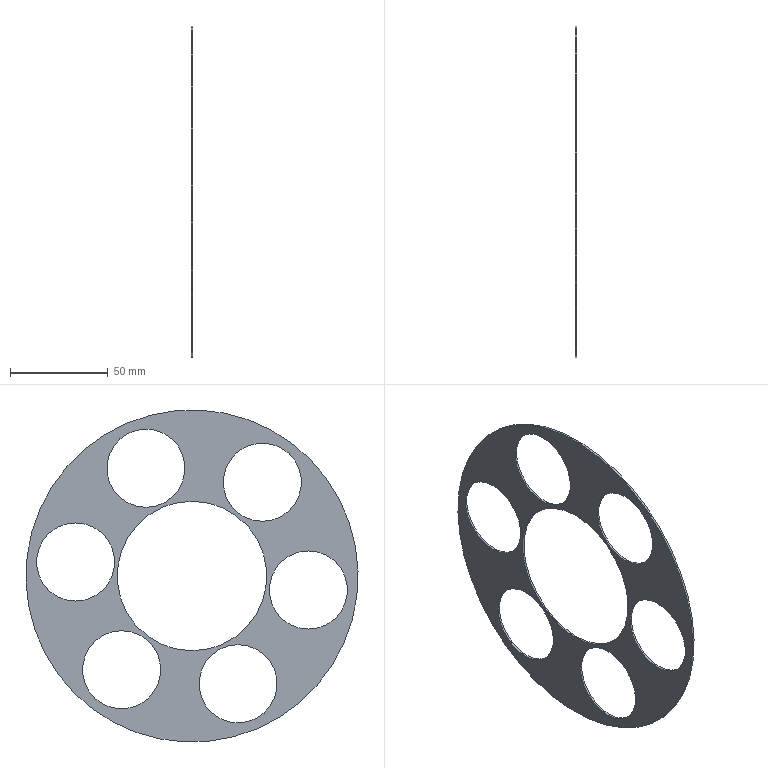Component | SolidWorks | 2018SOLIDWORKS1000000502-1 | 1 solid | 18 faces | box 1 x 170 x 170 mm | volume 10562 mm3 | cylinder 16 | plane 2 | commonest cylinder face diameters 40 x12 76.5 x2 170 x2 | material 201
STEP:
#1=COLOUR_RGB('',0.7922,0.8196,0.9333);
#2=FILL_AREA_STYLE_COLOUR('',#1);
#3=FILL_AREA_STYLE('',(#2));
#4=SURFACE_STYLE_FILL_AREA(#3);
#5=SURFACE_SIDE_STYLE('',(#4));
#6=SURFACE_STYLE_USAGE(.BOTH.,#5);
#7=PRESENTATION_STYLE_ASSIGNMENT((#6));
#8=CARTESIAN_POINT('',(0.3825,-4.408,10.134));
#9=VERTEX_POINT('',#8);
#10=CARTESIAN_POINT('',(0.3825,-5.972,9.946));
#11=VERTEX_POINT('',#10);
#12=CARTESIAN_POINT('',(0.3825,-5.19,10.04));
#13=DIRECTION('',(-1.,-0.,0.));
#14=DIRECTION('',(0.,-0.5999,0.8001));
#15=AXIS2_PLACEMENT_3D('',#12,#13,#14);
#16=CIRCLE('',#15,0.7874);
#17=EDGE_CURVE('',#9,#11,#16,.T.);
#18=ORIENTED_EDGE('',*,*,#17,.F.);
#19=CARTESIAN_POINT('',(0.3432,-4.408,10.134));
#20=VERTEX_POINT('',#19);
#21=CARTESIAN_POINT('',(0.3825,-4.408,10.134));
#22=DIRECTION('',(-1.,-0.,0.));
#23=VECTOR('',#22,39.37);
#24=LINE('',#21,#23);
#25=EDGE_CURVE('',#9,#20,#24,.T.);
#26=ORIENTED_EDGE('',*,*,#25,.T.);
#27=CARTESIAN_POINT('',(0.3432,-5.972,9.946));
#28=VERTEX_POINT('',#27);
#29=CARTESIAN_POINT('',(0.3432,-5.19,10.04));
#30=DIRECTION('',(-1.,-0.,0.));
#31=DIRECTION('',(0.,-0.5999,0.8001));
#32=AXIS2_PLACEMENT_3D('',#29,#30,#31);
#33=CIRCLE('',#32,0.7874);
#34=EDGE_CURVE('',#20,#28,#33,.T.);
#35=ORIENTED_EDGE('',*,*,#34,.T.);
#36=CARTESIAN_POINT('',(0.3825,-5.972,9.946));
#37=DIRECTION('',(-1.,-0.,0.));
#38=VECTOR('',#37,39.37);
#39=LINE('',#36,#38);
#40=EDGE_CURVE('',#11,#28,#39,.T.);
#41=ORIENTED_EDGE('',*,*,#40,.F.);
#42=EDGE_LOOP('',(#18,#26,#35,#41));
#43=FACE_OUTER_BOUND('',#42,.T.);
#44=CARTESIAN_POINT('',(0.3825,-5.19,10.04));
#45=DIRECTION('',(-1.,-0.,0.));
#46=DIRECTION('',(0.,-0.9928,-0.1195));
#47=AXIS2_PLACEMENT_3D('',#44,#45,#46);
#48=CYLINDRICAL_SURFACE('',#47,0.7874);
#49=ADVANCED_FACE('',(#43),#48,.F.);
#50=CARTESIAN_POINT('',(0.3825,-2.063,10.417));
#51=VERTEX_POINT('',#50);
#52=CARTESIAN_POINT('',(0.3825,-3.626,10.228));
#53=VERTEX_POINT('',#52);
#54=CARTESIAN_POINT('',(0.3825,-2.845,10.323));
#55=DIRECTION('',(-1.,-0.,0.));
#56=DIRECTION('',(0.,0.3929,0.9196));
#57=AXIS2_PLACEMENT_3D('',#54,#55,#56);
#58=CIRCLE('',#57,0.7874);
#59=EDGE_CURVE('',#51,#53,#58,.T.);
#60=ORIENTED_EDGE('',*,*,#59,.F.);
#61=CARTESIAN_POINT('',(0.3432,-2.063,10.417));
#62=VERTEX_POINT('',#61);
#63=CARTESIAN_POINT('',(0.3825,-2.063,10.417));
#64=DIRECTION('',(-1.,-0.,0.));
#65=VECTOR('',#64,39.37);
#66=LINE('',#63,#65);
#67=EDGE_CURVE('',#51,#62,#66,.T.);
#68=ORIENTED_EDGE('',*,*,#67,.T.);
#69=CARTESIAN_POINT('',(0.3432,-3.626,10.228));
#70=VERTEX_POINT('',#69);
#71=CARTESIAN_POINT('',(0.3432,-2.845,10.323));
#72=DIRECTION('',(-1.,-0.,0.));
#73=DIRECTION('',(0.,0.3929,0.9196));
#74=AXIS2_PLACEMENT_3D('',#71,#72,#73);
#75=CIRCLE('',#74,0.7874);
#76=EDGE_CURVE('',#62,#70,#75,.T.);
#77=ORIENTED_EDGE('',*,*,#76,.T.);
#78=CARTESIAN_POINT('',(0.3825,-3.626,10.228));
#79=DIRECTION('',(-1.,-0.,0.));
#80=VECTOR('',#79,39.37);
#81=LINE('',#78,#80);
#82=EDGE_CURVE('',#53,#70,#81,.T.);
#83=ORIENTED_EDGE('',*,*,#82,.F.);
#84=EDGE_LOOP('',(#60,#68,#77,#83));
#85=FACE_OUTER_BOUND('',#84,.T.);
#86=CARTESIAN_POINT('',(0.3825,-2.845,10.323));
#87=DIRECTION('',(-1.,-0.,0.));
#88=DIRECTION('',(0.,-0.9928,-0.1195));
#89=AXIS2_PLACEMENT_3D('',#86,#87,#88);
#90=CYLINDRICAL_SURFACE('',#89,0.7874);
#91=ADVANCED_FACE('',(#85),#90,.F.);
#92=CARTESIAN_POINT('',(0.3825,-0.6456,8.527));
#93=VERTEX_POINT('',#92);
#94=CARTESIAN_POINT('',(0.3825,-2.209,8.339));
#95=VERTEX_POINT('',#94);
#96=CARTESIAN_POINT('',(0.3825,-1.427,8.433));
#97=DIRECTION('',(-1.,-0.,0.));
#98=DIRECTION('',(-0.,0.9928,0.1195));
#99=AXIS2_PLACEMENT_3D('',#96,#97,#98);
#100=CIRCLE('',#99,0.7874);
#101=EDGE_CURVE('',#93,#95,#100,.T.);
#102=ORIENTED_EDGE('',*,*,#101,.F.);
#103=CARTESIAN_POINT('',(0.3432,-0.6456,8.527));
#104=VERTEX_POINT('',#103);
#105=CARTESIAN_POINT('',(0.3825,-0.6456,8.527));
#106=DIRECTION('',(-1.,-0.,0.));
#107=VECTOR('',#106,39.37);
#108=LINE('',#105,#107);
#109=EDGE_CURVE('',#93,#104,#108,.T.);
#110=ORIENTED_EDGE('',*,*,#109,.T.);
#111=CARTESIAN_POINT('',(0.3432,-2.209,8.339));
#112=VERTEX_POINT('',#111);
#113=CARTESIAN_POINT('',(0.3432,-1.427,8.433));
#114=DIRECTION('',(-1.,-0.,0.));
#115=DIRECTION('',(-0.,0.9928,0.1195));
#116=AXIS2_PLACEMENT_3D('',#113,#114,#115);
#117=CIRCLE('',#116,0.7874);
#118=EDGE_CURVE('',#104,#112,#117,.T.);
#119=ORIENTED_EDGE('',*,*,#118,.T.);
#120=CARTESIAN_POINT('',(0.3825,-2.209,8.339));
#121=DIRECTION('',(-1.,-0.,0.));
#122=VECTOR('',#121,39.37);
#123=LINE('',#120,#122);
#124=EDGE_CURVE('',#95,#112,#123,.T.);
#125=ORIENTED_EDGE('',*,*,#124,.F.);
#126=EDGE_LOOP('',(#102,#110,#119,#125));
#127=FACE_OUTER_BOUND('',#126,.T.);
#128=CARTESIAN_POINT('',(0.3825,-1.427,8.433));
#129=DIRECTION('',(-1.,-0.,0.));
#130=DIRECTION('',(0.,-0.9928,-0.1195));
#131=AXIS2_PLACEMENT_3D('',#128,#129,#130);
#132=CYLINDRICAL_SURFACE('',#131,0.7874);
#133=ADVANCED_FACE('',(#127),#132,.F.);
#134=CARTESIAN_POINT('',(0.3825,-1.574,6.355));
#135=VERTEX_POINT('',#134);
#136=CARTESIAN_POINT('',(0.3825,-3.137,6.166));
#137=VERTEX_POINT('',#136);
#138=CARTESIAN_POINT('',(0.3825,-2.355,6.26));
#139=DIRECTION('',(-1.,-0.,0.));
#140=DIRECTION('',(-0.,0.5999,-0.8001));
#141=AXIS2_PLACEMENT_3D('',#138,#139,#140);
#142=CIRCLE('',#141,0.7874);
#143=EDGE_CURVE('',#135,#137,#142,.T.);
#144=ORIENTED_EDGE('',*,*,#143,.F.);
#145=CARTESIAN_POINT('',(0.3432,-1.574,6.355));
#146=VERTEX_POINT('',#145);
#147=CARTESIAN_POINT('',(0.3825,-1.574,6.355));
#148=DIRECTION('',(-1.,-0.,0.));
#149=VECTOR('',#148,39.37);
#150=LINE('',#147,#149);
#151=EDGE_CURVE('',#135,#146,#150,.T.);
#152=ORIENTED_EDGE('',*,*,#151,.T.);
#153=CARTESIAN_POINT('',(0.3432,-3.137,6.166));
#154=VERTEX_POINT('',#153);
#155=CARTESIAN_POINT('',(0.3432,-2.355,6.26));
#156=DIRECTION('',(-1.,-0.,0.));
#157=DIRECTION('',(-0.,0.5999,-0.8001));
#158=AXIS2_PLACEMENT_3D('',#155,#156,#157);
#159=CIRCLE('',#158,0.7874);
#160=EDGE_CURVE('',#146,#154,#159,.T.);
#161=ORIENTED_EDGE('',*,*,#160,.T.);
#162=CARTESIAN_POINT('',(0.3825,-3.137,6.166));
#163=DIRECTION('',(-1.,-0.,0.));
#164=VECTOR('',#163,39.37);
#165=LINE('',#162,#164);
#166=EDGE_CURVE('',#137,#154,#165,.T.);
#167=ORIENTED_EDGE('',*,*,#166,.F.);
#168=EDGE_LOOP('',(#144,#152,#161,#167));
#169=FACE_OUTER_BOUND('',#168,.T.);
#170=CARTESIAN_POINT('',(0.3825,-2.355,6.26));
#171=DIRECTION('',(-1.,-0.,0.));
#172=DIRECTION('',(0.,-0.9928,-0.1195));
#173=AXIS2_PLACEMENT_3D('',#170,#171,#172);
#174=CYLINDRICAL_SURFACE('',#173,0.7874);
#175=ADVANCED_FACE('',(#169),#174,.F.);
#176=CARTESIAN_POINT('',(0.3825,-3.919,6.072));
#177=VERTEX_POINT('',#176);
#178=CARTESIAN_POINT('',(0.3825,-5.483,5.884));
#179=VERTEX_POINT('',#178);
#180=CARTESIAN_POINT('',(0.3825,-4.701,5.978));
#181=DIRECTION('',(-1.,-0.,0.));
#182=DIRECTION('',(-0.,-0.3929,-0.9196));
#183=AXIS2_PLACEMENT_3D('',#180,#181,#182);
#184=CIRCLE('',#183,0.7874);
#185=EDGE_CURVE('',#177,#179,#184,.T.);
#186=ORIENTED_EDGE('',*,*,#185,.F.);
#187=CARTESIAN_POINT('',(0.3432,-3.919,6.072));
#188=VERTEX_POINT('',#187);
#189=CARTESIAN_POINT('',(0.3825,-3.919,6.072));
#190=DIRECTION('',(-1.,-0.,0.));
#191=VECTOR('',#190,39.37);
#192=LINE('',#189,#191);
#193=EDGE_CURVE('',#177,#188,#192,.T.);
#194=ORIENTED_EDGE('',*,*,#193,.T.);
#195=CARTESIAN_POINT('',(0.3432,-5.483,5.884));
#196=VERTEX_POINT('',#195);
#197=CARTESIAN_POINT('',(0.3432,-4.701,5.978));
#198=DIRECTION('',(-1.,-0.,0.));
#199=DIRECTION('',(-0.,-0.3929,-0.9196));
#200=AXIS2_PLACEMENT_3D('',#197,#198,#199);
#201=CIRCLE('',#200,0.7874);
#202=EDGE_CURVE('',#188,#196,#201,.T.);
#203=ORIENTED_EDGE('',*,*,#202,.T.);
#204=CARTESIAN_POINT('',(0.3825,-5.483,5.884));
#205=DIRECTION('',(-1.,-0.,0.));
#206=VECTOR('',#205,39.37);
#207=LINE('',#204,#206);
#208=EDGE_CURVE('',#179,#196,#207,.T.);
#209=ORIENTED_EDGE('',*,*,#208,.F.);
#210=EDGE_LOOP('',(#186,#194,#203,#209));
#211=FACE_OUTER_BOUND('',#210,.T.);
#212=CARTESIAN_POINT('',(0.3825,-4.701,5.978));
#213=DIRECTION('',(-1.,-0.,0.));
#214=DIRECTION('',(0.,-0.9928,-0.1195));
#215=AXIS2_PLACEMENT_3D('',#212,#213,#214);
#216=CYLINDRICAL_SURFACE('',#215,0.7874);
#217=ADVANCED_FACE('',(#211),#216,.F.);
#218=CARTESIAN_POINT('',(0.3825,-5.336,7.962));
#219=VERTEX_POINT('',#218);
#220=CARTESIAN_POINT('',(0.3825,-6.9,7.774));
#221=VERTEX_POINT('',#220);
#222=CARTESIAN_POINT('',(0.3825,-6.118,7.868));
#223=DIRECTION('',(-1.,-0.,0.));
#224=DIRECTION('',(0.,-0.9928,-0.1195));
#225=AXIS2_PLACEMENT_3D('',#222,#223,#224);
#226=CIRCLE('',#225,0.7874);
#227=EDGE_CURVE('',#219,#221,#226,.T.);
#228=ORIENTED_EDGE('',*,*,#227,.F.);
#229=CARTESIAN_POINT('',(0.3432,-5.336,7.962));
#230=VERTEX_POINT('',#229);
#231=CARTESIAN_POINT('',(0.3825,-5.336,7.962));
#232=DIRECTION('',(-1.,-0.,0.));
#233=VECTOR('',#232,39.37);
#234=LINE('',#231,#233);
#235=EDGE_CURVE('',#219,#230,#234,.T.);
#236=ORIENTED_EDGE('',*,*,#235,.T.);
#237=CARTESIAN_POINT('',(0.3432,-6.9,7.774));
#238=VERTEX_POINT('',#237);
#239=CARTESIAN_POINT('',(0.3432,-6.118,7.868));
#240=DIRECTION('',(-1.,-0.,0.));
#241=DIRECTION('',(0.,-0.9928,-0.1195));
#242=AXIS2_PLACEMENT_3D('',#239,#240,#241);
#243=CIRCLE('',#242,0.7874);
#244=EDGE_CURVE('',#230,#238,#243,.T.);
#245=ORIENTED_EDGE('',*,*,#244,.T.);
#246=CARTESIAN_POINT('',(0.3825,-6.9,7.774));
#247=DIRECTION('',(-1.,-0.,0.));
#248=VECTOR('',#247,39.37);
#249=LINE('',#246,#248);
#250=EDGE_CURVE('',#221,#238,#249,.T.);
#251=ORIENTED_EDGE('',*,*,#250,.F.);
#252=EDGE_LOOP('',(#228,#236,#245,#251));
#253=FACE_OUTER_BOUND('',#252,.T.);
#254=CARTESIAN_POINT('',(0.3825,-6.118,7.868));
#255=DIRECTION('',(-1.,-0.,0.));
#256=DIRECTION('',(0.,-0.9928,-0.1195));
#257=AXIS2_PLACEMENT_3D('',#254,#255,#256);
#258=CYLINDRICAL_SURFACE('',#257,0.7874);
#259=ADVANCED_FACE('',(#253),#258,.F.);
#260=CARTESIAN_POINT('',(0.3825,-5.268,7.97));
#261=VERTEX_POINT('',#260);
#262=CARTESIAN_POINT('',(0.3825,-2.278,8.33));
#263=VERTEX_POINT('',#262);
#264=CARTESIAN_POINT('',(0.3825,-3.773,8.15));
#265=DIRECTION('',(1.,0.,-0.));
#266=DIRECTION('',(-0.,0.9928,0.1195));
#267=AXIS2_PLACEMENT_3D('',#264,#265,#266);
#268=CIRCLE('',#267,1.506);
#269=EDGE_CURVE('',#261,#263,#268,.T.);
#270=ORIENTED_EDGE('',*,*,#269,.T.);
#271=CARTESIAN_POINT('',(0.3432,-2.278,8.33));
#272=VERTEX_POINT('',#271);
#273=CARTESIAN_POINT('',(0.3825,-2.278,8.33));
#274=DIRECTION('',(-1.,-0.,0.));
#275=VECTOR('',#274,39.37);
#276=LINE('',#273,#275);
#277=EDGE_CURVE('',#263,#272,#276,.T.);
#278=ORIENTED_EDGE('',*,*,#277,.T.);
#279=CARTESIAN_POINT('',(0.3432,-5.268,7.97));
#280=VERTEX_POINT('',#279);
#281=CARTESIAN_POINT('',(0.3432,-3.773,8.15));
#282=DIRECTION('',(1.,0.,-0.));
#283=DIRECTION('',(-0.,0.9928,0.1195));
#284=AXIS2_PLACEMENT_3D('',#281,#282,#283);
#285=CIRCLE('',#284,1.506);
#286=EDGE_CURVE('',#280,#272,#285,.T.);
#287=ORIENTED_EDGE('',*,*,#286,.F.);
#288=CARTESIAN_POINT('',(0.3825,-5.268,7.97));
#289=DIRECTION('',(-1.,-0.,0.));
#290=VECTOR('',#289,39.37);
#291=LINE('',#288,#290);
#292=EDGE_CURVE('',#261,#280,#291,.T.);
#293=ORIENTED_EDGE('',*,*,#292,.F.);
#294=EDGE_LOOP('',(#270,#278,#287,#293));
#295=FACE_OUTER_BOUND('',#294,.T.);
#296=CARTESIAN_POINT('',(0.3825,-3.773,8.15));
#297=DIRECTION('',(-1.,-0.,0.));
#298=DIRECTION('',(0.,-0.9928,-0.1195));
#299=AXIS2_PLACEMENT_3D('',#296,#297,#298);
#300=CYLINDRICAL_SURFACE('',#299,1.506);
#301=ADVANCED_FACE('',(#295),#300,.F.);
#302=CARTESIAN_POINT('',(0.3825,-0.4502,8.55));
#303=VERTEX_POINT('',#302);
#304=CARTESIAN_POINT('',(0.3825,-7.095,7.75));
#305=VERTEX_POINT('',#304);
#306=CARTESIAN_POINT('',(0.3825,-3.773,8.15));
#307=DIRECTION('',(1.,0.,-0.));
#308=DIRECTION('',(-0.,0.9928,0.1195));
#309=AXIS2_PLACEMENT_3D('',#306,#307,#308);
#310=CIRCLE('',#309,3.346);
#311=EDGE_CURVE('',#303,#305,#310,.T.);
#312=ORIENTED_EDGE('',*,*,#311,.F.);
#313=CARTESIAN_POINT('',(0.3432,-0.4502,8.55));
#314=VERTEX_POINT('',#313);
#315=CARTESIAN_POINT('',(0.3825,-0.4502,8.55));
#316=DIRECTION('',(-1.,-0.,0.));
#317=VECTOR('',#316,39.37);
#318=LINE('',#315,#317);
#319=EDGE_CURVE('',#303,#314,#318,.T.);
#320=ORIENTED_EDGE('',*,*,#319,.T.);
#321=CARTESIAN_POINT('',(0.3432,-7.095,7.75));
#322=VERTEX_POINT('',#321);
#323=CARTESIAN_POINT('',(0.3432,-3.773,8.15));
#324=DIRECTION('',(1.,0.,-0.));
#325=DIRECTION('',(-0.,0.9928,0.1195));
#326=AXIS2_PLACEMENT_3D('',#323,#324,#325);
#327=CIRCLE('',#326,3.346);
#328=EDGE_CURVE('',#314,#322,#327,.T.);
#329=ORIENTED_EDGE('',*,*,#328,.T.);
#330=CARTESIAN_POINT('',(0.3825,-7.095,7.75));
#331=DIRECTION('',(-1.,-0.,0.));
#332=VECTOR('',#331,39.37);
#333=LINE('',#330,#332);
#334=EDGE_CURVE('',#305,#322,#333,.T.);
#335=ORIENTED_EDGE('',*,*,#334,.F.);
#336=EDGE_LOOP('',(#312,#320,#329,#335));
#337=FACE_OUTER_BOUND('',#336,.T.);
#338=CARTESIAN_POINT('',(0.3825,-3.773,8.15));
#339=DIRECTION('',(-1.,-0.,0.));
#340=DIRECTION('',(0.,-0.9928,-0.1195));
#341=AXIS2_PLACEMENT_3D('',#338,#339,#340);
#342=CYLINDRICAL_SURFACE('',#341,3.346);
#343=ADVANCED_FACE('',(#337),#342,.T.);
#344=CARTESIAN_POINT('',(0.3825,-5.19,10.04));
#345=DIRECTION('',(-1.,-0.,0.));
#346=DIRECTION('',(0.,-0.5999,0.8001));
#347=AXIS2_PLACEMENT_3D('',#344,#345,#346);
#348=CIRCLE('',#347,0.7874);
#349=EDGE_CURVE('',#11,#9,#348,.T.);
#350=ORIENTED_EDGE('',*,*,#349,.T.);
#351=ORIENTED_EDGE('',*,*,#17,.T.);
#352=EDGE_LOOP('',(#350,#351));
#353=FACE_BOUND('',#352,.T.);
#354=CARTESIAN_POINT('',(0.3825,-2.845,10.323));
#355=DIRECTION('',(-1.,-0.,0.));
#356=DIRECTION('',(0.,0.3929,0.9196));
#357=AXIS2_PLACEMENT_3D('',#354,#355,#356);
#358=CIRCLE('',#357,0.7874);
#359=EDGE_CURVE('',#53,#51,#358,.T.);
#360=ORIENTED_EDGE('',*,*,#359,.T.);
#361=ORIENTED_EDGE('',*,*,#59,.T.);
#362=EDGE_LOOP('',(#360,#361));
#363=FACE_BOUND('',#362,.T.);
#364=CARTESIAN_POINT('',(0.3825,-1.427,8.433));
#365=DIRECTION('',(-1.,-0.,0.));
#366=DIRECTION('',(-0.,0.9928,0.1195));
#367=AXIS2_PLACEMENT_3D('',#364,#365,#366);
#368=CIRCLE('',#367,0.7874);
#369=EDGE_CURVE('',#95,#93,#368,.T.);
#370=ORIENTED_EDGE('',*,*,#369,.T.);
#371=ORIENTED_EDGE('',*,*,#101,.T.);
#372=EDGE_LOOP('',(#370,#371));
#373=FACE_BOUND('',#372,.T.);
#374=CARTESIAN_POINT('',(0.3825,-2.355,6.26));
#375=DIRECTION('',(-1.,-0.,0.));
#376=DIRECTION('',(-0.,0.5999,-0.8001));
#377=AXIS2_PLACEMENT_3D('',#374,#375,#376);
#378=CIRCLE('',#377,0.7874);
#379=EDGE_CURVE('',#137,#135,#378,.T.);
#380=ORIENTED_EDGE('',*,*,#379,.T.);
#381=ORIENTED_EDGE('',*,*,#143,.T.);
#382=EDGE_LOOP('',(#380,#381));
#383=FACE_BOUND('',#382,.T.);
#384=CARTESIAN_POINT('',(0.3825,-4.701,5.978));
#385=DIRECTION('',(-1.,-0.,0.));
#386=DIRECTION('',(-0.,-0.3929,-0.9196));
#387=AXIS2_PLACEMENT_3D('',#384,#385,#386);
#388=CIRCLE('',#387,0.7874);
#389=EDGE_CURVE('',#179,#177,#388,.T.);
#390=ORIENTED_EDGE('',*,*,#389,.T.);
#391=ORIENTED_EDGE('',*,*,#185,.T.);
#392=EDGE_LOOP('',(#390,#391));
#393=FACE_BOUND('',#392,.T.);
#394=CARTESIAN_POINT('',(0.3825,-6.118,7.868));
#395=DIRECTION('',(-1.,-0.,0.));
#396=DIRECTION('',(0.,-0.9928,-0.1195));
#397=AXIS2_PLACEMENT_3D('',#394,#395,#396);
#398=CIRCLE('',#397,0.7874);
#399=EDGE_CURVE('',#221,#219,#398,.T.);
#400=ORIENTED_EDGE('',*,*,#399,.T.);
#401=ORIENTED_EDGE('',*,*,#227,.T.);
#402=EDGE_LOOP('',(#400,#401));
#403=FACE_BOUND('',#402,.T.);
#404=CARTESIAN_POINT('',(0.3825,-3.773,8.15));
#405=DIRECTION('',(1.,0.,-0.));
#406=DIRECTION('',(-0.,0.9928,0.1195));
#407=AXIS2_PLACEMENT_3D('',#404,#405,#406);
#408=CIRCLE('',#407,3.346);
#409=EDGE_CURVE('',#305,#303,#408,.T.);
#410=ORIENTED_EDGE('',*,*,#409,.T.);
#411=ORIENTED_EDGE('',*,*,#311,.T.);
#412=EDGE_LOOP('',(#410,#411));
#413=FACE_OUTER_BOUND('',#412,.T.);
#414=ORIENTED_EDGE('',*,*,#269,.F.);
#415=CARTESIAN_POINT('',(0.3825,-3.773,8.15));
#416=DIRECTION('',(1.,0.,-0.));
#417=DIRECTION('',(-0.,0.9928,0.1195));
#418=AXIS2_PLACEMENT_3D('',#415,#416,#417);
#419=CIRCLE('',#418,1.506);
#420=EDGE_CURVE('',#263,#261,#419,.T.);
#421=ORIENTED_EDGE('',*,*,#420,.F.);
#422=EDGE_LOOP('',(#414,#421));
#423=FACE_BOUND('',#422,.T.);
#424=CARTESIAN_POINT('',(0.3825,-3.773,8.15));
#425=DIRECTION('',(1.,0.,-0.));
#426=DIRECTION('',(-0.,0.9928,0.1195));
#427=AXIS2_PLACEMENT_3D('',#424,#425,#426);
#428=PLANE('',#427);
#429=ADVANCED_FACE('',(#353,#363,#373,#383,#393,#403,#413,#423),#428,.T.);
#430=CARTESIAN_POINT('',(0.3432,-5.19,10.04));
#431=DIRECTION('',(-1.,-0.,0.));
#432=DIRECTION('',(0.,-0.5999,0.8001));
#433=AXIS2_PLACEMENT_3D('',#430,#431,#432);
#434=CIRCLE('',#433,0.7874);
#435=EDGE_CURVE('',#28,#20,#434,.T.);
#436=ORIENTED_EDGE('',*,*,#435,.F.);
#437=ORIENTED_EDGE('',*,*,#34,.F.);
#438=EDGE_LOOP('',(#436,#437));
#439=FACE_BOUND('',#438,.T.);
#440=CARTESIAN_POINT('',(0.3432,-2.845,10.323));
#441=DIRECTION('',(-1.,-0.,0.));
#442=DIRECTION('',(0.,0.3929,0.9196));
#443=AXIS2_PLACEMENT_3D('',#440,#441,#442);
#444=CIRCLE('',#443,0.7874);
#445=EDGE_CURVE('',#70,#62,#444,.T.);
#446=ORIENTED_EDGE('',*,*,#445,.F.);
#447=ORIENTED_EDGE('',*,*,#76,.F.);
#448=EDGE_LOOP('',(#446,#447));
#449=FACE_BOUND('',#448,.T.);
#450=CARTESIAN_POINT('',(0.3432,-1.427,8.433));
#451=DIRECTION('',(-1.,-0.,0.));
#452=DIRECTION('',(-0.,0.9928,0.1195));
#453=AXIS2_PLACEMENT_3D('',#450,#451,#452);
#454=CIRCLE('',#453,0.7874);
#455=EDGE_CURVE('',#112,#104,#454,.T.);
#456=ORIENTED_EDGE('',*,*,#455,.F.);
#457=ORIENTED_EDGE('',*,*,#118,.F.);
#458=EDGE_LOOP('',(#456,#457));
#459=FACE_BOUND('',#458,.T.);
#460=CARTESIAN_POINT('',(0.3432,-2.355,6.26));
#461=DIRECTION('',(-1.,-0.,0.));
#462=DIRECTION('',(-0.,0.5999,-0.8001));
#463=AXIS2_PLACEMENT_3D('',#460,#461,#462);
#464=CIRCLE('',#463,0.7874);
#465=EDGE_CURVE('',#154,#146,#464,.T.);
#466=ORIENTED_EDGE('',*,*,#465,.F.);
#467=ORIENTED_EDGE('',*,*,#160,.F.);
#468=EDGE_LOOP('',(#466,#467));
#469=FACE_BOUND('',#468,.T.);
#470=CARTESIAN_POINT('',(0.3432,-4.701,5.978));
#471=DIRECTION('',(-1.,-0.,0.));
#472=DIRECTION('',(-0.,-0.3929,-0.9196));
#473=AXIS2_PLACEMENT_3D('',#470,#471,#472);
#474=CIRCLE('',#473,0.7874);
#475=EDGE_CURVE('',#196,#188,#474,.T.);
#476=ORIENTED_EDGE('',*,*,#475,.F.);
#477=ORIENTED_EDGE('',*,*,#202,.F.);
#478=EDGE_LOOP('',(#476,#477));
#479=FACE_BOUND('',#478,.T.);
#480=CARTESIAN_POINT('',(0.3432,-6.118,7.868));
#481=DIRECTION('',(-1.,-0.,0.));
#482=DIRECTION('',(0.,-0.9928,-0.1195));
#483=AXIS2_PLACEMENT_3D('',#480,#481,#482);
#484=CIRCLE('',#483,0.7874);
#485=EDGE_CURVE('',#238,#230,#484,.T.);
#486=ORIENTED_EDGE('',*,*,#485,.F.);
#487=ORIENTED_EDGE('',*,*,#244,.F.);
#488=EDGE_LOOP('',(#486,#487));
#489=FACE_BOUND('',#488,.T.);
#490=CARTESIAN_POINT('',(0.3432,-3.773,8.15));
#491=DIRECTION('',(1.,0.,-0.));
#492=DIRECTION('',(-0.,0.9928,0.1195));
#493=AXIS2_PLACEMENT_3D('',#490,#491,#492);
#494=CIRCLE('',#493,3.346);
#495=EDGE_CURVE('',#322,#314,#494,.T.);
#496=ORIENTED_EDGE('',*,*,#495,.F.);
#497=ORIENTED_EDGE('',*,*,#328,.F.);
#498=EDGE_LOOP('',(#496,#497));
#499=FACE_OUTER_BOUND('',#498,.T.);
#500=ORIENTED_EDGE('',*,*,#286,.T.);
#501=CARTESIAN_POINT('',(0.3432,-3.773,8.15));
#502=DIRECTION('',(1.,0.,-0.));
#503=DIRECTION('',(-0.,0.9928,0.1195));
#504=AXIS2_PLACEMENT_3D('',#501,#502,#503);
#505=CIRCLE('',#504,1.506);
#506=EDGE_CURVE('',#272,#280,#505,.T.);
#507=ORIENTED_EDGE('',*,*,#506,.T.);
#508=EDGE_LOOP('',(#500,#507));
#509=FACE_BOUND('',#508,.T.);
#510=CARTESIAN_POINT('',(0.3432,-3.773,8.15));
#511=DIRECTION('',(1.,0.,-0.));
#512=DIRECTION('',(-0.,0.9928,0.1195));
#513=AXIS2_PLACEMENT_3D('',#510,#511,#512);
#514=PLANE('',#513);
#515=ADVANCED_FACE('',(#439,#449,#459,#469,#479,#489,#499,#509),#514,.F.);
#516=ORIENTED_EDGE('',*,*,#319,.F.);
#517=ORIENTED_EDGE('',*,*,#409,.F.);
#518=ORIENTED_EDGE('',*,*,#334,.T.);
#519=ORIENTED_EDGE('',*,*,#495,.T.);
#520=EDGE_LOOP('',(#516,#517,#518,#519));
#521=FACE_OUTER_BOUND('',#520,.T.);
#522=CARTESIAN_POINT('',(0.3825,-3.773,8.15));
#523=DIRECTION('',(-1.,-0.,0.));
#524=DIRECTION('',(0.,-0.9928,-0.1195));
#525=AXIS2_PLACEMENT_3D('',#522,#523,#524);
#526=CYLINDRICAL_SURFACE('',#525,3.346);
#527=ADVANCED_FACE('',(#521),#526,.T.);
#528=ORIENTED_EDGE('',*,*,#277,.F.);
#529=ORIENTED_EDGE('',*,*,#420,.T.);
#530=ORIENTED_EDGE('',*,*,#292,.T.);
#531=ORIENTED_EDGE('',*,*,#506,.F.);
#532=EDGE_LOOP('',(#528,#529,#530,#531));
#533=FACE_OUTER_BOUND('',#532,.T.);
#534=CARTESIAN_POINT('',(0.3825,-3.773,8.15));
#535=DIRECTION('',(-1.,-0.,0.));
#536=DIRECTION('',(0.,-0.9928,-0.1195));
#537=AXIS2_PLACEMENT_3D('',#534,#535,#536);
#538=CYLINDRICAL_SURFACE('',#537,1.506);
#539=ADVANCED_FACE('',(#533),#538,.F.);
#540=ORIENTED_EDGE('',*,*,#235,.F.);
#541=ORIENTED_EDGE('',*,*,#399,.F.);
#542=ORIENTED_EDGE('',*,*,#250,.T.);
#543=ORIENTED_EDGE('',*,*,#485,.T.);
#544=EDGE_LOOP('',(#540,#541,#542,#543));
#545=FACE_OUTER_BOUND('',#544,.T.);
#546=CARTESIAN_POINT('',(0.3825,-6.118,7.868));
#547=DIRECTION('',(-1.,-0.,0.));
#548=DIRECTION('',(0.,-0.9928,-0.1195));
#549=AXIS2_PLACEMENT_3D('',#546,#547,#548);
#550=CYLINDRICAL_SURFACE('',#549,0.7874);
#551=ADVANCED_FACE('',(#545),#550,.F.);
#552=ORIENTED_EDGE('',*,*,#193,.F.);
#553=ORIENTED_EDGE('',*,*,#389,.F.);
#554=ORIENTED_EDGE('',*,*,#208,.T.);
#555=ORIENTED_EDGE('',*,*,#475,.T.);
#556=EDGE_LOOP('',(#552,#553,#554,#555));
#557=FACE_OUTER_BOUND('',#556,.T.);
#558=CARTESIAN_POINT('',(0.3825,-4.701,5.978));
#559=DIRECTION('',(-1.,-0.,0.));
#560=DIRECTION('',(0.,-0.9928,-0.1195));
#561=AXIS2_PLACEMENT_3D('',#558,#559,#560);
#562=CYLINDRICAL_SURFACE('',#561,0.7874);
#563=ADVANCED_FACE('',(#557),#562,.F.);
#564=ORIENTED_EDGE('',*,*,#151,.F.);
#565=ORIENTED_EDGE('',*,*,#379,.F.);
#566=ORIENTED_EDGE('',*,*,#166,.T.);
#567=ORIENTED_EDGE('',*,*,#465,.T.);
#568=EDGE_LOOP('',(#564,#565,#566,#567));
#569=FACE_OUTER_BOUND('',#568,.T.);
#570=CARTESIAN_POINT('',(0.3825,-2.355,6.26));
#571=DIRECTION('',(-1.,-0.,0.));
#572=DIRECTION('',(0.,-0.9928,-0.1195));
#573=AXIS2_PLACEMENT_3D('',#570,#571,#572);
#574=CYLINDRICAL_SURFACE('',#573,0.7874);
#575=ADVANCED_FACE('',(#569),#574,.F.);
#576=ORIENTED_EDGE('',*,*,#109,.F.);
#577=ORIENTED_EDGE('',*,*,#369,.F.);
#578=ORIENTED_EDGE('',*,*,#124,.T.);
#579=ORIENTED_EDGE('',*,*,#455,.T.);
#580=EDGE_LOOP('',(#576,#577,#578,#579));
#581=FACE_OUTER_BOUND('',#580,.T.);
#582=CARTESIAN_POINT('',(0.3825,-1.427,8.433));
#583=DIRECTION('',(-1.,-0.,0.));
#584=DIRECTION('',(0.,-0.9928,-0.1195));
#585=AXIS2_PLACEMENT_3D('',#582,#583,#584);
#586=CYLINDRICAL_SURFACE('',#585,0.7874);
#587=ADVANCED_FACE('',(#581),#586,.F.);
#588=ORIENTED_EDGE('',*,*,#67,.F.);
#589=ORIENTED_EDGE('',*,*,#359,.F.);
#590=ORIENTED_EDGE('',*,*,#82,.T.);
#591=ORIENTED_EDGE('',*,*,#445,.T.);
#592=EDGE_LOOP('',(#588,#589,#590,#591));
#593=FACE_OUTER_BOUND('',#592,.T.);
#594=CARTESIAN_POINT('',(0.3825,-2.845,10.323));
#595=DIRECTION('',(-1.,-0.,0.));
#596=DIRECTION('',(0.,-0.9928,-0.1195));
#597=AXIS2_PLACEMENT_3D('',#594,#595,#596);
#598=CYLINDRICAL_SURFACE('',#597,0.7874);
#599=ADVANCED_FACE('',(#593),#598,.F.);
#600=ORIENTED_EDGE('',*,*,#25,.F.);
#601=ORIENTED_EDGE('',*,*,#349,.F.);
#602=ORIENTED_EDGE('',*,*,#40,.T.);
#603=ORIENTED_EDGE('',*,*,#435,.T.);
#604=EDGE_LOOP('',(#600,#601,#602,#603));
#605=FACE_OUTER_BOUND('',#604,.T.);
#606=CARTESIAN_POINT('',(0.3825,-5.19,10.04));
#607=DIRECTION('',(-1.,-0.,0.));
#608=DIRECTION('',(0.,-0.9928,-0.1195));
#609=AXIS2_PLACEMENT_3D('',#606,#607,#608);
#610=CYLINDRICAL_SURFACE('',#609,0.7874);
#611=ADVANCED_FACE('',(#605),#610,.F.);
#612=CLOSED_SHELL('',(#49,#91,#133,#175,#217,#259,#301,#343,#429,#515,#527,#539,#551,#563,#575,#587,#599,#611));
#613=MANIFOLD_SOLID_BREP('',#612);
#614=STYLED_ITEM('',(#7),#613);
#615=PRESENTATION_LAYER_ASSIGNMENT('','',(#614));
#616=CARTESIAN_POINT('',(0.,0.,0.));
#617=DIRECTION('',(0.,0.,1.));
#618=DIRECTION('',(1.,0.,0.));
#619=AXIS2_PLACEMENT_3D('',#616,#617,#618);
#620=(LENGTH_UNIT()NAMED_UNIT(*)SI_UNIT($,.METRE.));
#621=LENGTH_MEASURE_WITH_UNIT(LENGTH_MEASURE(0.0254),#620);
#622=DIMENSIONAL_EXPONENTS(1.,0.,0.,0.,0.,0.,0.);
#623=(CONVERSION_BASED_UNIT('',#621)LENGTH_UNIT()NAMED_UNIT(#622));
#624=UNCERTAINTY_MEASURE_WITH_UNIT(LENGTH_MEASURE(0.00001),#623,'','');
#625=(NAMED_UNIT(*)PLANE_ANGLE_UNIT()SI_UNIT($,.RADIAN.));
#626=(NAMED_UNIT(*)SI_UNIT($,.STERADIAN.)SOLID_ANGLE_UNIT());
#627=(GEOMETRIC_REPRESENTATION_CONTEXT(3)GLOBAL_UNCERTAINTY_ASSIGNED_CONTEXT((#624))GLOBAL_UNIT_ASSIGNED_CONTEXT((#623,#625,#626))REPRESENTATION_CONTEXT('',''));
#628=ADVANCED_BREP_SHAPE_REPRESENTATION('',(#613,#619),#627);
#629=(LENGTH_UNIT()NAMED_UNIT(*)SI_UNIT($,.METRE.));
#630=LENGTH_MEASURE_WITH_UNIT(LENGTH_MEASURE(0.0254),#629);
#631=DIMENSIONAL_EXPONENTS(1.,0.,0.,0.,0.,0.,0.);
#632=(CONVERSION_BASED_UNIT('',#630)LENGTH_UNIT()NAMED_UNIT(#631));
#633=UNCERTAINTY_MEASURE_WITH_UNIT(LENGTH_MEASURE(0.00001),#632,'','');
#634=(NAMED_UNIT(*)PLANE_ANGLE_UNIT()SI_UNIT($,.RADIAN.));
#635=(NAMED_UNIT(*)SI_UNIT($,.STERADIAN.)SOLID_ANGLE_UNIT());
#636=(GEOMETRIC_REPRESENTATION_CONTEXT(3)GLOBAL_UNCERTAINTY_ASSIGNED_CONTEXT((#633))GLOBAL_UNIT_ASSIGNED_CONTEXT((#632,#634,#635))REPRESENTATION_CONTEXT('',''));
#637=MECHANICAL_DESIGN_GEOMETRIC_PRESENTATION_REPRESENTATION('',(#614),#636);